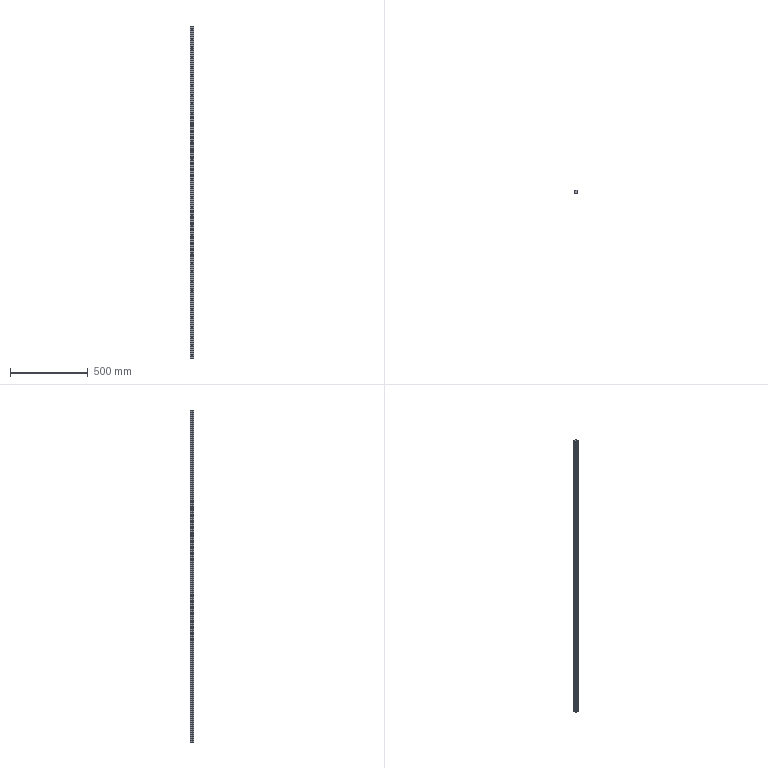Component | SolidWorks | HG_RAIL0_R_ANY_1-2 | 1 solid | 214 faces | volume 892657 mm3 | cylinder 148 | plane 66 | commonest cylinder face diameters 11 x72 7 x72 4.6 x4